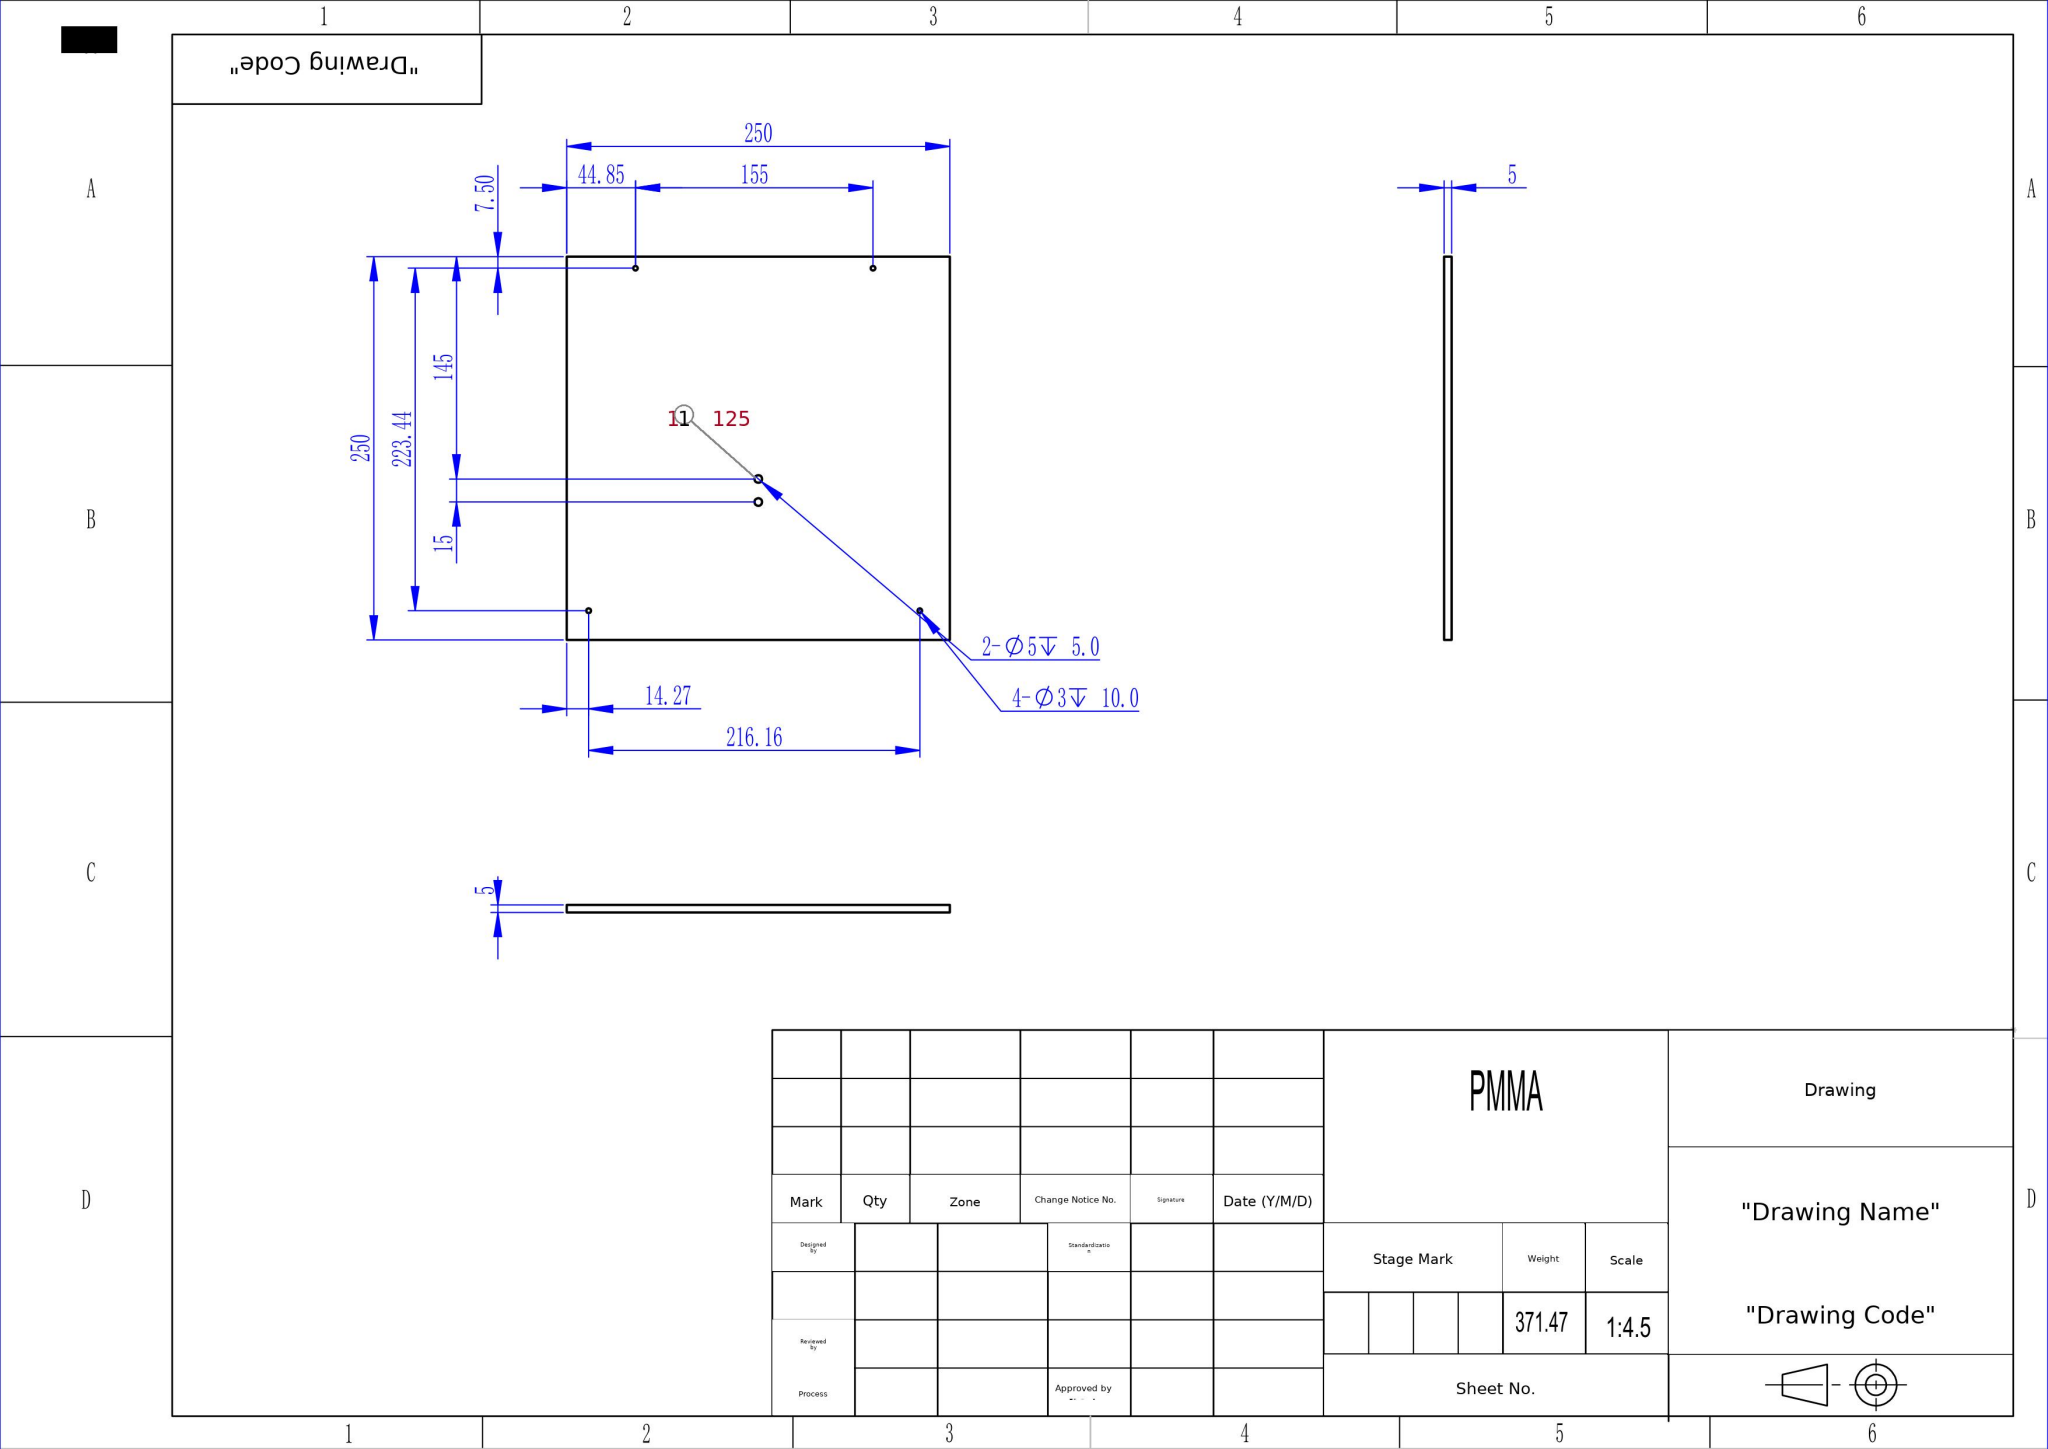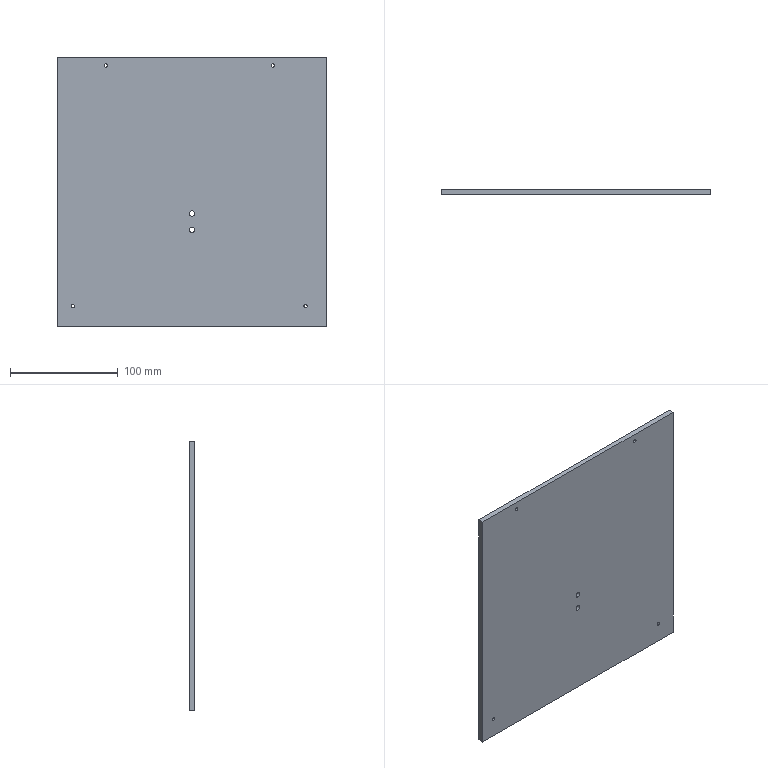Part | SolidWorks | mm | material PMMA | 1 solid | 18 faces | box 250 x 5 x 250 mm | volume 312162 mm3 | cylinder 12 | plane 6 | commonest cylinder face diameters 3 x8 5 x4
build123d program:
from build123d import *

# Parameters (mm, degrees)
SKETCH1_W           = 250
SKETCH1_H           = 250
BOSS_EXTRUDE1_DEPTH = 5
SKETCH2_R           = 2.5
CUT_EXTRUDE1_DEPTH  = 5
SKETCH3_R           = 1.5
CUT_EXTRUDE2_DEPTH  = 10


with BuildPart() as part:
    # Sketch1 → Boss-Extrude1 (new body)
    with BuildSketch(Plane(origin=(0, 0, 0), x_dir=(1, 0, 0), z_dir=(0, 1, 0))):
        Rectangle(SKETCH1_W, SKETCH1_H)
    extrude(amount=BOSS_EXTRUDE1_DEPTH)

    # Sketch2 → Cut-Extrude1 (cut)
    with BuildSketch(Plane(origin=(0, 5, 0), x_dir=(1, 0, 0), z_dir=(0, 1, 0))):
        with Locations(Location((0, 35, 0), (0, 0, 270))):
            Circle(SKETCH2_R)
        with Locations(Location((0, 20, 0), (0, 0, 270))):
            Circle(SKETCH2_R)
    extrude(amount=-CUT_EXTRUDE1_DEPTH, mode=Mode.SUBTRACT)

    # Sketch3 → Cut-Extrude2 (cut)
    with BuildSketch(Plane(origin=(0, 5, 0), x_dir=(1, 0, 0), z_dir=(0, 1, 0))):
        with Locations(Location((74.854, -117.5, 0), (0, 0, 270))):
            Circle(SKETCH3_R)
        with Locations(Location((-80.146, -117.5, 0), (0, 0, 270))):
            Circle(SKETCH3_R)
        with Locations(Location((-110.728, 105.936, 0), (0, 0, 270))):
            Circle(SKETCH3_R)
        with Locations(Location((105.435, 105.936, 0), (0, 0, 270))):
            Circle(SKETCH3_R)
    extrude(amount=-CUT_EXTRUDE2_DEPTH, mode=Mode.SUBTRACT)


solid = part.part
STEP:
#1=CARTESIAN_POINT('',(105.435,0.,-107.436));
#2=VERTEX_POINT('',#1);
#3=CARTESIAN_POINT('',(105.435,0.,-104.436));
#4=VERTEX_POINT('',#3);
#5=CARTESIAN_POINT('',(105.435,0.,-105.936));
#6=DIRECTION('',(0.,1.,0.));
#7=DIRECTION('',(0.,0.,1.));
#8=AXIS2_PLACEMENT_3D('',#5,#6,#7);
#9=CIRCLE('',#8,1.5);
#10=EDGE_CURVE('',#2,#4,#9,.T.);
#11=ORIENTED_EDGE('',*,*,#10,.F.);
#12=CARTESIAN_POINT('',(105.435,5.,-107.436));
#13=VERTEX_POINT('',#12);
#14=CARTESIAN_POINT('',(105.435,-5.,-107.436));
#15=DIRECTION('',(0.,1.,0.));
#16=VECTOR('',#15,1000.);
#17=LINE('',#14,#16);
#18=EDGE_CURVE('',#2,#13,#17,.T.);
#19=ORIENTED_EDGE('',*,*,#18,.T.);
#20=CARTESIAN_POINT('',(105.435,5.,-104.436));
#21=VERTEX_POINT('',#20);
#22=CARTESIAN_POINT('',(105.435,5.,-105.936));
#23=DIRECTION('',(0.,1.,0.));
#24=DIRECTION('',(0.,0.,1.));
#25=AXIS2_PLACEMENT_3D('',#22,#23,#24);
#26=CIRCLE('',#25,1.5);
#27=EDGE_CURVE('',#13,#21,#26,.T.);
#28=ORIENTED_EDGE('',*,*,#27,.T.);
#29=CARTESIAN_POINT('',(105.435,-5.,-104.436));
#30=DIRECTION('',(0.,1.,0.));
#31=VECTOR('',#30,1000.);
#32=LINE('',#29,#31);
#33=EDGE_CURVE('',#4,#21,#32,.T.);
#34=ORIENTED_EDGE('',*,*,#33,.F.);
#35=EDGE_LOOP('',(#11,#19,#28,#34));
#36=FACE_OUTER_BOUND('',#35,.T.);
#37=CARTESIAN_POINT('',(105.435,-5.,-105.936));
#38=DIRECTION('',(0.,1.,0.));
#39=DIRECTION('',(0.,0.,1.));
#40=AXIS2_PLACEMENT_3D('',#37,#38,#39);
#41=CYLINDRICAL_SURFACE('',#40,1.5);
#42=ADVANCED_FACE('',(#36),#41,.F.);
#43=CARTESIAN_POINT('',(-110.728,0.,-107.436));
#44=VERTEX_POINT('',#43);
#45=CARTESIAN_POINT('',(-110.728,0.,-104.436));
#46=VERTEX_POINT('',#45);
#47=CARTESIAN_POINT('',(-110.728,0.,-105.936));
#48=DIRECTION('',(0.,1.,0.));
#49=DIRECTION('',(0.,0.,1.));
#50=AXIS2_PLACEMENT_3D('',#47,#48,#49);
#51=CIRCLE('',#50,1.5);
#52=EDGE_CURVE('',#44,#46,#51,.T.);
#53=ORIENTED_EDGE('',*,*,#52,.F.);
#54=CARTESIAN_POINT('',(-110.728,5.,-107.436));
#55=VERTEX_POINT('',#54);
#56=CARTESIAN_POINT('',(-110.728,-5.,-107.436));
#57=DIRECTION('',(0.,1.,0.));
#58=VECTOR('',#57,1000.);
#59=LINE('',#56,#58);
#60=EDGE_CURVE('',#44,#55,#59,.T.);
#61=ORIENTED_EDGE('',*,*,#60,.T.);
#62=CARTESIAN_POINT('',(-110.728,5.,-104.436));
#63=VERTEX_POINT('',#62);
#64=CARTESIAN_POINT('',(-110.728,5.,-105.936));
#65=DIRECTION('',(0.,1.,0.));
#66=DIRECTION('',(0.,0.,1.));
#67=AXIS2_PLACEMENT_3D('',#64,#65,#66);
#68=CIRCLE('',#67,1.5);
#69=EDGE_CURVE('',#55,#63,#68,.T.);
#70=ORIENTED_EDGE('',*,*,#69,.T.);
#71=CARTESIAN_POINT('',(-110.728,-5.,-104.436));
#72=DIRECTION('',(0.,1.,0.));
#73=VECTOR('',#72,1000.);
#74=LINE('',#71,#73);
#75=EDGE_CURVE('',#46,#63,#74,.T.);
#76=ORIENTED_EDGE('',*,*,#75,.F.);
#77=EDGE_LOOP('',(#53,#61,#70,#76));
#78=FACE_OUTER_BOUND('',#77,.T.);
#79=CARTESIAN_POINT('',(-110.728,-5.,-105.936));
#80=DIRECTION('',(0.,1.,0.));
#81=DIRECTION('',(0.,0.,1.));
#82=AXIS2_PLACEMENT_3D('',#79,#80,#81);
#83=CYLINDRICAL_SURFACE('',#82,1.5);
#84=ADVANCED_FACE('',(#78),#83,.F.);
#85=CARTESIAN_POINT('',(-80.146,0.,116.));
#86=VERTEX_POINT('',#85);
#87=CARTESIAN_POINT('',(-80.146,0.,119.));
#88=VERTEX_POINT('',#87);
#89=CARTESIAN_POINT('',(-80.146,0.,117.5));
#90=DIRECTION('',(0.,1.,0.));
#91=DIRECTION('',(0.,0.,1.));
#92=AXIS2_PLACEMENT_3D('',#89,#90,#91);
#93=CIRCLE('',#92,1.5);
#94=EDGE_CURVE('',#86,#88,#93,.T.);
#95=ORIENTED_EDGE('',*,*,#94,.F.);
#96=CARTESIAN_POINT('',(-80.146,5.,116.));
#97=VERTEX_POINT('',#96);
#98=CARTESIAN_POINT('',(-80.146,-5.,116.));
#99=DIRECTION('',(0.,1.,0.));
#100=VECTOR('',#99,1000.);
#101=LINE('',#98,#100);
#102=EDGE_CURVE('',#86,#97,#101,.T.);
#103=ORIENTED_EDGE('',*,*,#102,.T.);
#104=CARTESIAN_POINT('',(-80.146,5.,119.));
#105=VERTEX_POINT('',#104);
#106=CARTESIAN_POINT('',(-80.146,5.,117.5));
#107=DIRECTION('',(0.,1.,0.));
#108=DIRECTION('',(0.,0.,1.));
#109=AXIS2_PLACEMENT_3D('',#106,#107,#108);
#110=CIRCLE('',#109,1.5);
#111=EDGE_CURVE('',#97,#105,#110,.T.);
#112=ORIENTED_EDGE('',*,*,#111,.T.);
#113=CARTESIAN_POINT('',(-80.146,-5.,119.));
#114=DIRECTION('',(0.,1.,0.));
#115=VECTOR('',#114,1000.);
#116=LINE('',#113,#115);
#117=EDGE_CURVE('',#88,#105,#116,.T.);
#118=ORIENTED_EDGE('',*,*,#117,.F.);
#119=EDGE_LOOP('',(#95,#103,#112,#118));
#120=FACE_OUTER_BOUND('',#119,.T.);
#121=CARTESIAN_POINT('',(-80.146,-5.,117.5));
#122=DIRECTION('',(0.,1.,0.));
#123=DIRECTION('',(0.,0.,1.));
#124=AXIS2_PLACEMENT_3D('',#121,#122,#123);
#125=CYLINDRICAL_SURFACE('',#124,1.5);
#126=ADVANCED_FACE('',(#120),#125,.F.);
#127=CARTESIAN_POINT('',(74.854,0.,116.));
#128=VERTEX_POINT('',#127);
#129=CARTESIAN_POINT('',(74.854,0.,119.));
#130=VERTEX_POINT('',#129);
#131=CARTESIAN_POINT('',(74.854,0.,117.5));
#132=DIRECTION('',(0.,1.,0.));
#133=DIRECTION('',(0.,0.,1.));
#134=AXIS2_PLACEMENT_3D('',#131,#132,#133);
#135=CIRCLE('',#134,1.5);
#136=EDGE_CURVE('',#128,#130,#135,.T.);
#137=ORIENTED_EDGE('',*,*,#136,.F.);
#138=CARTESIAN_POINT('',(74.854,5.,116.));
#139=VERTEX_POINT('',#138);
#140=CARTESIAN_POINT('',(74.854,-5.,116.));
#141=DIRECTION('',(0.,1.,0.));
#142=VECTOR('',#141,1000.);
#143=LINE('',#140,#142);
#144=EDGE_CURVE('',#128,#139,#143,.T.);
#145=ORIENTED_EDGE('',*,*,#144,.T.);
#146=CARTESIAN_POINT('',(74.854,5.,119.));
#147=VERTEX_POINT('',#146);
#148=CARTESIAN_POINT('',(74.854,5.,117.5));
#149=DIRECTION('',(0.,1.,0.));
#150=DIRECTION('',(0.,0.,1.));
#151=AXIS2_PLACEMENT_3D('',#148,#149,#150);
#152=CIRCLE('',#151,1.5);
#153=EDGE_CURVE('',#139,#147,#152,.T.);
#154=ORIENTED_EDGE('',*,*,#153,.T.);
#155=CARTESIAN_POINT('',(74.854,-5.,119.));
#156=DIRECTION('',(0.,1.,0.));
#157=VECTOR('',#156,1000.);
#158=LINE('',#155,#157);
#159=EDGE_CURVE('',#130,#147,#158,.T.);
#160=ORIENTED_EDGE('',*,*,#159,.F.);
#161=EDGE_LOOP('',(#137,#145,#154,#160));
#162=FACE_OUTER_BOUND('',#161,.T.);
#163=CARTESIAN_POINT('',(74.854,-5.,117.5));
#164=DIRECTION('',(0.,1.,0.));
#165=DIRECTION('',(0.,0.,1.));
#166=AXIS2_PLACEMENT_3D('',#163,#164,#165);
#167=CYLINDRICAL_SURFACE('',#166,1.5);
#168=ADVANCED_FACE('',(#162),#167,.F.);
#169=CARTESIAN_POINT('',(0.,0.,-37.5));
#170=VERTEX_POINT('',#169);
#171=CARTESIAN_POINT('',(0.,0.,-32.5));
#172=VERTEX_POINT('',#171);
#173=CARTESIAN_POINT('',(0.,0.,-35.));
#174=DIRECTION('',(0.,1.,0.));
#175=DIRECTION('',(0.,0.,1.));
#176=AXIS2_PLACEMENT_3D('',#173,#174,#175);
#177=CIRCLE('',#176,2.5);
#178=EDGE_CURVE('',#170,#172,#177,.T.);
#179=ORIENTED_EDGE('',*,*,#178,.F.);
#180=CARTESIAN_POINT('',(0.,5.,-37.5));
#181=VERTEX_POINT('',#180);
#182=CARTESIAN_POINT('',(0.,0.,-37.5));
#183=DIRECTION('',(0.,1.,0.));
#184=VECTOR('',#183,1000.);
#185=LINE('',#182,#184);
#186=EDGE_CURVE('',#170,#181,#185,.T.);
#187=ORIENTED_EDGE('',*,*,#186,.T.);
#188=CARTESIAN_POINT('',(0.,5.,-32.5));
#189=VERTEX_POINT('',#188);
#190=CARTESIAN_POINT('',(0.,5.,-35.));
#191=DIRECTION('',(0.,1.,0.));
#192=DIRECTION('',(0.,0.,1.));
#193=AXIS2_PLACEMENT_3D('',#190,#191,#192);
#194=CIRCLE('',#193,2.5);
#195=EDGE_CURVE('',#181,#189,#194,.T.);
#196=ORIENTED_EDGE('',*,*,#195,.T.);
#197=CARTESIAN_POINT('',(0.,0.,-32.5));
#198=DIRECTION('',(0.,1.,0.));
#199=VECTOR('',#198,1000.);
#200=LINE('',#197,#199);
#201=EDGE_CURVE('',#172,#189,#200,.T.);
#202=ORIENTED_EDGE('',*,*,#201,.F.);
#203=EDGE_LOOP('',(#179,#187,#196,#202));
#204=FACE_OUTER_BOUND('',#203,.T.);
#205=CARTESIAN_POINT('',(0.,0.,-35.));
#206=DIRECTION('',(0.,1.,0.));
#207=DIRECTION('',(0.,0.,1.));
#208=AXIS2_PLACEMENT_3D('',#205,#206,#207);
#209=CYLINDRICAL_SURFACE('',#208,2.5);
#210=ADVANCED_FACE('',(#204),#209,.F.);
#211=CARTESIAN_POINT('',(0.,0.,-22.5));
#212=VERTEX_POINT('',#211);
#213=CARTESIAN_POINT('',(0.,0.,-17.5));
#214=VERTEX_POINT('',#213);
#215=CARTESIAN_POINT('',(0.,0.,-20.));
#216=DIRECTION('',(0.,1.,0.));
#217=DIRECTION('',(0.,0.,1.));
#218=AXIS2_PLACEMENT_3D('',#215,#216,#217);
#219=CIRCLE('',#218,2.5);
#220=EDGE_CURVE('',#212,#214,#219,.T.);
#221=ORIENTED_EDGE('',*,*,#220,.F.);
#222=CARTESIAN_POINT('',(0.,5.,-22.5));
#223=VERTEX_POINT('',#222);
#224=CARTESIAN_POINT('',(0.,0.,-22.5));
#225=DIRECTION('',(0.,1.,0.));
#226=VECTOR('',#225,1000.);
#227=LINE('',#224,#226);
#228=EDGE_CURVE('',#212,#223,#227,.T.);
#229=ORIENTED_EDGE('',*,*,#228,.T.);
#230=CARTESIAN_POINT('',(0.,5.,-17.5));
#231=VERTEX_POINT('',#230);
#232=CARTESIAN_POINT('',(0.,5.,-20.));
#233=DIRECTION('',(0.,1.,0.));
#234=DIRECTION('',(0.,0.,1.));
#235=AXIS2_PLACEMENT_3D('',#232,#233,#234);
#236=CIRCLE('',#235,2.5);
#237=EDGE_CURVE('',#223,#231,#236,.T.);
#238=ORIENTED_EDGE('',*,*,#237,.T.);
#239=CARTESIAN_POINT('',(0.,0.,-17.5));
#240=DIRECTION('',(0.,1.,0.));
#241=VECTOR('',#240,1000.);
#242=LINE('',#239,#241);
#243=EDGE_CURVE('',#214,#231,#242,.T.);
#244=ORIENTED_EDGE('',*,*,#243,.F.);
#245=EDGE_LOOP('',(#221,#229,#238,#244));
#246=FACE_OUTER_BOUND('',#245,.T.);
#247=CARTESIAN_POINT('',(0.,0.,-20.));
#248=DIRECTION('',(0.,1.,0.));
#249=DIRECTION('',(0.,0.,1.));
#250=AXIS2_PLACEMENT_3D('',#247,#248,#249);
#251=CYLINDRICAL_SURFACE('',#250,2.5);
#252=ADVANCED_FACE('',(#246),#251,.F.);
#253=CARTESIAN_POINT('',(125.,0.,125.));
#254=VERTEX_POINT('',#253);
#255=CARTESIAN_POINT('',(125.,0.,-125.));
#256=VERTEX_POINT('',#255);
#257=CARTESIAN_POINT('',(125.,0.,-125.));
#258=DIRECTION('',(0.,0.,-1.));
#259=VECTOR('',#258,1000.);
#260=LINE('',#257,#259);
#261=EDGE_CURVE('',#254,#256,#260,.T.);
#262=ORIENTED_EDGE('',*,*,#261,.T.);
#263=CARTESIAN_POINT('',(125.,5.,-125.));
#264=VERTEX_POINT('',#263);
#265=CARTESIAN_POINT('',(125.,5.,-125.));
#266=DIRECTION('',(0.,-1.,0.));
#267=VECTOR('',#266,1000.);
#268=LINE('',#265,#267);
#269=EDGE_CURVE('',#264,#256,#268,.T.);
#270=ORIENTED_EDGE('',*,*,#269,.F.);
#271=CARTESIAN_POINT('',(125.,5.,125.));
#272=VERTEX_POINT('',#271);
#273=CARTESIAN_POINT('',(125.,5.,-125.));
#274=DIRECTION('',(0.,0.,-1.));
#275=VECTOR('',#274,1000.);
#276=LINE('',#273,#275);
#277=EDGE_CURVE('',#272,#264,#276,.T.);
#278=ORIENTED_EDGE('',*,*,#277,.F.);
#279=CARTESIAN_POINT('',(125.,5.,125.));
#280=DIRECTION('',(0.,-1.,0.));
#281=VECTOR('',#280,1000.);
#282=LINE('',#279,#281);
#283=EDGE_CURVE('',#272,#254,#282,.T.);
#284=ORIENTED_EDGE('',*,*,#283,.T.);
#285=EDGE_LOOP('',(#262,#270,#278,#284));
#286=FACE_OUTER_BOUND('',#285,.T.);
#287=CARTESIAN_POINT('',(125.,5.,-125.));
#288=DIRECTION('',(-1.,0.,0.));
#289=DIRECTION('',(0.,0.,1.));
#290=AXIS2_PLACEMENT_3D('',#287,#288,#289);
#291=PLANE('',#290);
#292=ADVANCED_FACE('',(#286),#291,.F.);
#293=CARTESIAN_POINT('',(-125.,0.,-125.));
#294=VERTEX_POINT('',#293);
#295=CARTESIAN_POINT('',(-125.,0.,-125.));
#296=DIRECTION('',(-1.,0.,0.));
#297=VECTOR('',#296,1000.);
#298=LINE('',#295,#297);
#299=EDGE_CURVE('',#256,#294,#298,.T.);
#300=ORIENTED_EDGE('',*,*,#299,.T.);
#301=CARTESIAN_POINT('',(-125.,5.,-125.));
#302=VERTEX_POINT('',#301);
#303=CARTESIAN_POINT('',(-125.,5.,-125.));
#304=DIRECTION('',(0.,-1.,0.));
#305=VECTOR('',#304,1000.);
#306=LINE('',#303,#305);
#307=EDGE_CURVE('',#302,#294,#306,.T.);
#308=ORIENTED_EDGE('',*,*,#307,.F.);
#309=CARTESIAN_POINT('',(-125.,5.,-125.));
#310=DIRECTION('',(-1.,0.,0.));
#311=VECTOR('',#310,1000.);
#312=LINE('',#309,#311);
#313=EDGE_CURVE('',#264,#302,#312,.T.);
#314=ORIENTED_EDGE('',*,*,#313,.F.);
#315=ORIENTED_EDGE('',*,*,#269,.T.);
#316=EDGE_LOOP('',(#300,#308,#314,#315));
#317=FACE_OUTER_BOUND('',#316,.T.);
#318=CARTESIAN_POINT('',(-125.,5.,-125.));
#319=DIRECTION('',(0.,0.,1.));
#320=DIRECTION('',(1.,0.,0.));
#321=AXIS2_PLACEMENT_3D('',#318,#319,#320);
#322=PLANE('',#321);
#323=ADVANCED_FACE('',(#317),#322,.F.);
#324=CARTESIAN_POINT('',(-125.,0.,125.));
#325=VERTEX_POINT('',#324);
#326=CARTESIAN_POINT('',(-125.,0.,-125.));
#327=DIRECTION('',(0.,0.,1.));
#328=VECTOR('',#327,1000.);
#329=LINE('',#326,#328);
#330=EDGE_CURVE('',#294,#325,#329,.T.);
#331=ORIENTED_EDGE('',*,*,#330,.T.);
#332=CARTESIAN_POINT('',(-125.,5.,125.));
#333=VERTEX_POINT('',#332);
#334=CARTESIAN_POINT('',(-125.,5.,125.));
#335=DIRECTION('',(0.,-1.,0.));
#336=VECTOR('',#335,1000.);
#337=LINE('',#334,#336);
#338=EDGE_CURVE('',#333,#325,#337,.T.);
#339=ORIENTED_EDGE('',*,*,#338,.F.);
#340=CARTESIAN_POINT('',(-125.,5.,-125.));
#341=DIRECTION('',(0.,0.,1.));
#342=VECTOR('',#341,1000.);
#343=LINE('',#340,#342);
#344=EDGE_CURVE('',#302,#333,#343,.T.);
#345=ORIENTED_EDGE('',*,*,#344,.F.);
#346=ORIENTED_EDGE('',*,*,#307,.T.);
#347=EDGE_LOOP('',(#331,#339,#345,#346));
#348=FACE_OUTER_BOUND('',#347,.T.);
#349=CARTESIAN_POINT('',(-125.,5.,-125.));
#350=DIRECTION('',(1.,0.,-0.));
#351=DIRECTION('',(-0.,0.,-1.));
#352=AXIS2_PLACEMENT_3D('',#349,#350,#351);
#353=PLANE('',#352);
#354=ADVANCED_FACE('',(#348),#353,.F.);
#355=CARTESIAN_POINT('',(-125.,0.,125.));
#356=DIRECTION('',(1.,0.,0.));
#357=VECTOR('',#356,1000.);
#358=LINE('',#355,#357);
#359=EDGE_CURVE('',#325,#254,#358,.T.);
#360=ORIENTED_EDGE('',*,*,#359,.T.);
#361=ORIENTED_EDGE('',*,*,#283,.F.);
#362=CARTESIAN_POINT('',(-125.,5.,125.));
#363=DIRECTION('',(1.,0.,0.));
#364=VECTOR('',#363,1000.);
#365=LINE('',#362,#364);
#366=EDGE_CURVE('',#333,#272,#365,.T.);
#367=ORIENTED_EDGE('',*,*,#366,.F.);
#368=ORIENTED_EDGE('',*,*,#338,.T.);
#369=EDGE_LOOP('',(#360,#361,#367,#368));
#370=FACE_OUTER_BOUND('',#369,.T.);
#371=CARTESIAN_POINT('',(-125.,5.,125.));
#372=DIRECTION('',(0.,0.,-1.));
#373=DIRECTION('',(-1.,0.,0.));
#374=AXIS2_PLACEMENT_3D('',#371,#372,#373);
#375=PLANE('',#374);
#376=ADVANCED_FACE('',(#370),#375,.F.);
#377=CARTESIAN_POINT('',(105.435,5.,-105.936));
#378=DIRECTION('',(0.,1.,0.));
#379=DIRECTION('',(0.,0.,1.));
#380=AXIS2_PLACEMENT_3D('',#377,#378,#379);
#381=CIRCLE('',#380,1.5);
#382=EDGE_CURVE('',#21,#13,#381,.T.);
#383=ORIENTED_EDGE('',*,*,#382,.F.);
#384=ORIENTED_EDGE('',*,*,#27,.F.);
#385=EDGE_LOOP('',(#383,#384));
#386=FACE_BOUND('',#385,.T.);
#387=CARTESIAN_POINT('',(-110.728,5.,-105.936));
#388=DIRECTION('',(0.,1.,0.));
#389=DIRECTION('',(0.,0.,1.));
#390=AXIS2_PLACEMENT_3D('',#387,#388,#389);
#391=CIRCLE('',#390,1.5);
#392=EDGE_CURVE('',#63,#55,#391,.T.);
#393=ORIENTED_EDGE('',*,*,#392,.F.);
#394=ORIENTED_EDGE('',*,*,#69,.F.);
#395=EDGE_LOOP('',(#393,#394));
#396=FACE_BOUND('',#395,.T.);
#397=CARTESIAN_POINT('',(-80.146,5.,117.5));
#398=DIRECTION('',(0.,1.,0.));
#399=DIRECTION('',(0.,0.,1.));
#400=AXIS2_PLACEMENT_3D('',#397,#398,#399);
#401=CIRCLE('',#400,1.5);
#402=EDGE_CURVE('',#105,#97,#401,.T.);
#403=ORIENTED_EDGE('',*,*,#402,.F.);
#404=ORIENTED_EDGE('',*,*,#111,.F.);
#405=EDGE_LOOP('',(#403,#404));
#406=FACE_BOUND('',#405,.T.);
#407=CARTESIAN_POINT('',(74.854,5.,117.5));
#408=DIRECTION('',(0.,1.,0.));
#409=DIRECTION('',(0.,0.,1.));
#410=AXIS2_PLACEMENT_3D('',#407,#408,#409);
#411=CIRCLE('',#410,1.5);
#412=EDGE_CURVE('',#147,#139,#411,.T.);
#413=ORIENTED_EDGE('',*,*,#412,.F.);
#414=ORIENTED_EDGE('',*,*,#153,.F.);
#415=EDGE_LOOP('',(#413,#414));
#416=FACE_BOUND('',#415,.T.);
#417=CARTESIAN_POINT('',(0.,5.,-35.));
#418=DIRECTION('',(0.,1.,0.));
#419=DIRECTION('',(0.,0.,1.));
#420=AXIS2_PLACEMENT_3D('',#417,#418,#419);
#421=CIRCLE('',#420,2.5);
#422=EDGE_CURVE('',#189,#181,#421,.T.);
#423=ORIENTED_EDGE('',*,*,#422,.F.);
#424=ORIENTED_EDGE('',*,*,#195,.F.);
#425=EDGE_LOOP('',(#423,#424));
#426=FACE_BOUND('',#425,.T.);
#427=CARTESIAN_POINT('',(0.,5.,-20.));
#428=DIRECTION('',(0.,1.,0.));
#429=DIRECTION('',(0.,0.,1.));
#430=AXIS2_PLACEMENT_3D('',#427,#428,#429);
#431=CIRCLE('',#430,2.5);
#432=EDGE_CURVE('',#231,#223,#431,.T.);
#433=ORIENTED_EDGE('',*,*,#432,.F.);
#434=ORIENTED_EDGE('',*,*,#237,.F.);
#435=EDGE_LOOP('',(#433,#434));
#436=FACE_BOUND('',#435,.T.);
#437=ORIENTED_EDGE('',*,*,#277,.T.);
#438=ORIENTED_EDGE('',*,*,#313,.T.);
#439=ORIENTED_EDGE('',*,*,#344,.T.);
#440=ORIENTED_EDGE('',*,*,#366,.T.);
#441=EDGE_LOOP('',(#437,#438,#439,#440));
#442=FACE_OUTER_BOUND('',#441,.T.);
#443=CARTESIAN_POINT('',(0.,5.,0.));
#444=DIRECTION('',(0.,1.,0.));
#445=DIRECTION('',(0.,0.,1.));
#446=AXIS2_PLACEMENT_3D('',#443,#444,#445);
#447=PLANE('',#446);
#448=ADVANCED_FACE('',(#386,#396,#406,#416,#426,#436,#442),#447,.T.);
#449=CARTESIAN_POINT('',(105.435,0.,-105.936));
#450=DIRECTION('',(0.,1.,0.));
#451=DIRECTION('',(0.,0.,1.));
#452=AXIS2_PLACEMENT_3D('',#449,#450,#451);
#453=CIRCLE('',#452,1.5);
#454=EDGE_CURVE('',#4,#2,#453,.T.);
#455=ORIENTED_EDGE('',*,*,#454,.T.);
#456=ORIENTED_EDGE('',*,*,#10,.T.);
#457=EDGE_LOOP('',(#455,#456));
#458=FACE_BOUND('',#457,.T.);
#459=CARTESIAN_POINT('',(-110.728,0.,-105.936));
#460=DIRECTION('',(0.,1.,0.));
#461=DIRECTION('',(0.,0.,1.));
#462=AXIS2_PLACEMENT_3D('',#459,#460,#461);
#463=CIRCLE('',#462,1.5);
#464=EDGE_CURVE('',#46,#44,#463,.T.);
#465=ORIENTED_EDGE('',*,*,#464,.T.);
#466=ORIENTED_EDGE('',*,*,#52,.T.);
#467=EDGE_LOOP('',(#465,#466));
#468=FACE_BOUND('',#467,.T.);
#469=CARTESIAN_POINT('',(-80.146,0.,117.5));
#470=DIRECTION('',(0.,1.,0.));
#471=DIRECTION('',(0.,0.,1.));
#472=AXIS2_PLACEMENT_3D('',#469,#470,#471);
#473=CIRCLE('',#472,1.5);
#474=EDGE_CURVE('',#88,#86,#473,.T.);
#475=ORIENTED_EDGE('',*,*,#474,.T.);
#476=ORIENTED_EDGE('',*,*,#94,.T.);
#477=EDGE_LOOP('',(#475,#476));
#478=FACE_BOUND('',#477,.T.);
#479=CARTESIAN_POINT('',(74.854,0.,117.5));
#480=DIRECTION('',(0.,1.,0.));
#481=DIRECTION('',(0.,0.,1.));
#482=AXIS2_PLACEMENT_3D('',#479,#480,#481);
#483=CIRCLE('',#482,1.5);
#484=EDGE_CURVE('',#130,#128,#483,.T.);
#485=ORIENTED_EDGE('',*,*,#484,.T.);
#486=ORIENTED_EDGE('',*,*,#136,.T.);
#487=EDGE_LOOP('',(#485,#486));
#488=FACE_BOUND('',#487,.T.);
#489=CARTESIAN_POINT('',(0.,0.,-35.));
#490=DIRECTION('',(0.,1.,0.));
#491=DIRECTION('',(0.,0.,1.));
#492=AXIS2_PLACEMENT_3D('',#489,#490,#491);
#493=CIRCLE('',#492,2.5);
#494=EDGE_CURVE('',#172,#170,#493,.T.);
#495=ORIENTED_EDGE('',*,*,#494,.T.);
#496=ORIENTED_EDGE('',*,*,#178,.T.);
#497=EDGE_LOOP('',(#495,#496));
#498=FACE_BOUND('',#497,.T.);
#499=CARTESIAN_POINT('',(0.,0.,-20.));
#500=DIRECTION('',(0.,1.,0.));
#501=DIRECTION('',(0.,0.,1.));
#502=AXIS2_PLACEMENT_3D('',#499,#500,#501);
#503=CIRCLE('',#502,2.5);
#504=EDGE_CURVE('',#214,#212,#503,.T.);
#505=ORIENTED_EDGE('',*,*,#504,.T.);
#506=ORIENTED_EDGE('',*,*,#220,.T.);
#507=EDGE_LOOP('',(#505,#506));
#508=FACE_BOUND('',#507,.T.);
#509=ORIENTED_EDGE('',*,*,#261,.F.);
#510=ORIENTED_EDGE('',*,*,#359,.F.);
#511=ORIENTED_EDGE('',*,*,#330,.F.);
#512=ORIENTED_EDGE('',*,*,#299,.F.);
#513=EDGE_LOOP('',(#509,#510,#511,#512));
#514=FACE_OUTER_BOUND('',#513,.T.);
#515=CARTESIAN_POINT('',(0.,0.,0.));
#516=DIRECTION('',(0.,1.,0.));
#517=DIRECTION('',(0.,0.,1.));
#518=AXIS2_PLACEMENT_3D('',#515,#516,#517);
#519=PLANE('',#518);
#520=ADVANCED_FACE('',(#458,#468,#478,#488,#498,#508,#514),#519,.F.);
#521=ORIENTED_EDGE('',*,*,#228,.F.);
#522=ORIENTED_EDGE('',*,*,#504,.F.);
#523=ORIENTED_EDGE('',*,*,#243,.T.);
#524=ORIENTED_EDGE('',*,*,#432,.T.);
#525=EDGE_LOOP('',(#521,#522,#523,#524));
#526=FACE_OUTER_BOUND('',#525,.T.);
#527=CARTESIAN_POINT('',(0.,0.,-20.));
#528=DIRECTION('',(0.,1.,0.));
#529=DIRECTION('',(0.,0.,1.));
#530=AXIS2_PLACEMENT_3D('',#527,#528,#529);
#531=CYLINDRICAL_SURFACE('',#530,2.5);
#532=ADVANCED_FACE('',(#526),#531,.F.);
#533=ORIENTED_EDGE('',*,*,#186,.F.);
#534=ORIENTED_EDGE('',*,*,#494,.F.);
#535=ORIENTED_EDGE('',*,*,#201,.T.);
#536=ORIENTED_EDGE('',*,*,#422,.T.);
#537=EDGE_LOOP('',(#533,#534,#535,#536));
#538=FACE_OUTER_BOUND('',#537,.T.);
#539=CARTESIAN_POINT('',(0.,0.,-35.));
#540=DIRECTION('',(0.,1.,0.));
#541=DIRECTION('',(0.,0.,1.));
#542=AXIS2_PLACEMENT_3D('',#539,#540,#541);
#543=CYLINDRICAL_SURFACE('',#542,2.5);
#544=ADVANCED_FACE('',(#538),#543,.F.);
#545=ORIENTED_EDGE('',*,*,#144,.F.);
#546=ORIENTED_EDGE('',*,*,#484,.F.);
#547=ORIENTED_EDGE('',*,*,#159,.T.);
#548=ORIENTED_EDGE('',*,*,#412,.T.);
#549=EDGE_LOOP('',(#545,#546,#547,#548));
#550=FACE_OUTER_BOUND('',#549,.T.);
#551=CARTESIAN_POINT('',(74.854,-5.,117.5));
#552=DIRECTION('',(0.,1.,0.));
#553=DIRECTION('',(0.,0.,1.));
#554=AXIS2_PLACEMENT_3D('',#551,#552,#553);
#555=CYLINDRICAL_SURFACE('',#554,1.5);
#556=ADVANCED_FACE('',(#550),#555,.F.);
#557=ORIENTED_EDGE('',*,*,#102,.F.);
#558=ORIENTED_EDGE('',*,*,#474,.F.);
#559=ORIENTED_EDGE('',*,*,#117,.T.);
#560=ORIENTED_EDGE('',*,*,#402,.T.);
#561=EDGE_LOOP('',(#557,#558,#559,#560));
#562=FACE_OUTER_BOUND('',#561,.T.);
#563=CARTESIAN_POINT('',(-80.146,-5.,117.5));
#564=DIRECTION('',(0.,1.,0.));
#565=DIRECTION('',(0.,0.,1.));
#566=AXIS2_PLACEMENT_3D('',#563,#564,#565);
#567=CYLINDRICAL_SURFACE('',#566,1.5);
#568=ADVANCED_FACE('',(#562),#567,.F.);
#569=ORIENTED_EDGE('',*,*,#60,.F.);
#570=ORIENTED_EDGE('',*,*,#464,.F.);
#571=ORIENTED_EDGE('',*,*,#75,.T.);
#572=ORIENTED_EDGE('',*,*,#392,.T.);
#573=EDGE_LOOP('',(#569,#570,#571,#572));
#574=FACE_OUTER_BOUND('',#573,.T.);
#575=CARTESIAN_POINT('',(-110.728,-5.,-105.936));
#576=DIRECTION('',(0.,1.,0.));
#577=DIRECTION('',(0.,0.,1.));
#578=AXIS2_PLACEMENT_3D('',#575,#576,#577);
#579=CYLINDRICAL_SURFACE('',#578,1.5);
#580=ADVANCED_FACE('',(#574),#579,.F.);
#581=ORIENTED_EDGE('',*,*,#18,.F.);
#582=ORIENTED_EDGE('',*,*,#454,.F.);
#583=ORIENTED_EDGE('',*,*,#33,.T.);
#584=ORIENTED_EDGE('',*,*,#382,.T.);
#585=EDGE_LOOP('',(#581,#582,#583,#584));
#586=FACE_OUTER_BOUND('',#585,.T.);
#587=CARTESIAN_POINT('',(105.435,-5.,-105.936));
#588=DIRECTION('',(0.,1.,0.));
#589=DIRECTION('',(0.,0.,1.));
#590=AXIS2_PLACEMENT_3D('',#587,#588,#589);
#591=CYLINDRICAL_SURFACE('',#590,1.5);
#592=ADVANCED_FACE('',(#586),#591,.F.);
#593=CLOSED_SHELL('',(#42,#84,#126,#168,#210,#252,#292,#323,#354,#376,#448,#520,#532,#544,#556,#568,#580,#592));
#594=MANIFOLD_SOLID_BREP('',#593);
#595=CARTESIAN_POINT('',(0.,0.,0.));
#596=DIRECTION('',(0.,0.,1.));
#597=DIRECTION('',(1.,0.,0.));
#598=AXIS2_PLACEMENT_3D('',#595,#596,#597);
#599=(LENGTH_UNIT()NAMED_UNIT(*)SI_UNIT(.MILLI.,.METRE.));
#600=UNCERTAINTY_MEASURE_WITH_UNIT(LENGTH_MEASURE(0.00001),#599,'','');
#601=(NAMED_UNIT(*)PLANE_ANGLE_UNIT()SI_UNIT($,.RADIAN.));
#602=(NAMED_UNIT(*)SI_UNIT($,.STERADIAN.)SOLID_ANGLE_UNIT());
#603=(GEOMETRIC_REPRESENTATION_CONTEXT(3)GLOBAL_UNCERTAINTY_ASSIGNED_CONTEXT((#600))GLOBAL_UNIT_ASSIGNED_CONTEXT((#599,#601,#602))REPRESENTATION_CONTEXT('',''));
#604=ADVANCED_BREP_SHAPE_REPRESENTATION('',(#594,#598),#603);